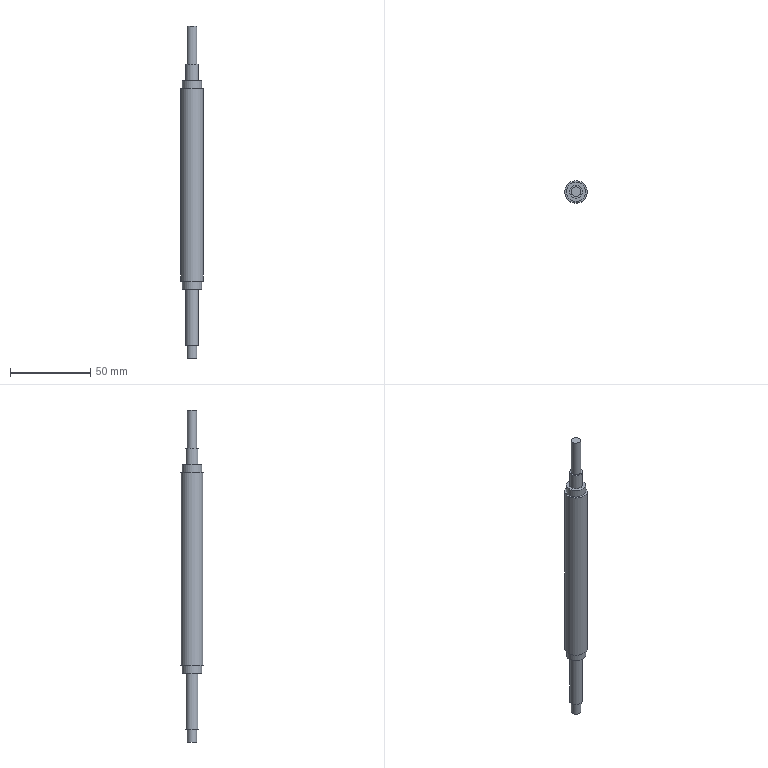Component | NX | Z_AXIS_LEADSCREW | 1 solid | 15 faces | box 14 x 14 x 207 mm | volume 22770 mm3 | plane 8 | cylinder 7 | commonest cylinder face diameters 6 x2 8 x2 12 x2 14 x1
STEP:
#1=CARTESIAN_POINT('',(0.,0.,0.));
#2=DIRECTION('',(0.,0.,1.));
#3=DIRECTION('',(1.,0.,0.));
#4=AXIS2_PLACEMENT_3D('',#1,#2,#3);
#5=CARTESIAN_POINT('',(628.689,-150.302,-1191.));
#6=VERTEX_POINT('',#5);
#7=CARTESIAN_POINT('',(625.689,-150.302,-1191.));
#8=DIRECTION('',(0.,0.,1.));
#9=DIRECTION('',(1.,0.,0.));
#10=AXIS2_PLACEMENT_3D('',#7,#8,#9);
#11=CIRCLE('',#10,3.);
#12=CARTESIAN_POINT('',(625.689,-150.302,-1191.));
#13=DIRECTION('',(0.,0.,1.));
#14=DIRECTION('',(1.,0.,0.));
#15=AXIS2_PLACEMENT_3D('',#12,#13,#14);
#16=PLANE('',#15);
#17=CARTESIAN_POINT('',(0.,0.));
#18=DIRECTION('',(1.,0.));
#19=AXIS2_PLACEMENT_2D('',#17,#18);
#20=CIRCLE('',#19,3.);
#21=(GEOMETRIC_REPRESENTATION_CONTEXT(2)PARAMETRIC_REPRESENTATION_CONTEXT()REPRESENTATION_CONTEXT('',''));
#22=DEFINITIONAL_REPRESENTATION('',(#20),#21);
#23=PCURVE('',#16,#22);
#24=CARTESIAN_POINT('',(625.689,-150.302,-1083.));
#25=DIRECTION('',(0.,0.,1.));
#26=DIRECTION('',(1.,0.,0.));
#27=AXIS2_PLACEMENT_3D('',#24,#25,#26);
#28=CYLINDRICAL_SURFACE('',#27,3.);
#29=CARTESIAN_POINT('',(0.,-108.));
#30=DIRECTION('',(1.,0.));
#31=VECTOR('',#30,1.);
#32=LINE('',#29,#31);
#33=(GEOMETRIC_REPRESENTATION_CONTEXT(2)PARAMETRIC_REPRESENTATION_CONTEXT()REPRESENTATION_CONTEXT('',''));
#34=DEFINITIONAL_REPRESENTATION('',(#32),#33);
#35=PCURVE('',#28,#34);
#36=SURFACE_CURVE('',#11,(#23,#35),.PCURVE_S1.);
#37=EDGE_CURVE('',#6,#6,#36,.T.);
#38=ORIENTED_EDGE('',*,*,#37,.F.);
#39=EDGE_LOOP('',(#38));
#40=FACE_BOUND('',#39,.T.);
#41=ADVANCED_FACE('',(#40),#16,.F.);
#42=CARTESIAN_POINT('',(628.689,-150.302,-984.));
#43=VERTEX_POINT('',#42);
#44=CARTESIAN_POINT('',(625.689,-150.302,-984.));
#45=DIRECTION('',(0.,0.,1.));
#46=DIRECTION('',(1.,0.,0.));
#47=AXIS2_PLACEMENT_3D('',#44,#45,#46);
#48=CIRCLE('',#47,3.);
#49=CARTESIAN_POINT('',(625.689,-150.302,-984.));
#50=DIRECTION('',(0.,0.,1.));
#51=DIRECTION('',(1.,0.,0.));
#52=AXIS2_PLACEMENT_3D('',#49,#50,#51);
#53=PLANE('',#52);
#54=CARTESIAN_POINT('',(0.,0.));
#55=DIRECTION('',(1.,0.));
#56=AXIS2_PLACEMENT_2D('',#54,#55);
#57=CIRCLE('',#56,3.);
#58=(GEOMETRIC_REPRESENTATION_CONTEXT(2)PARAMETRIC_REPRESENTATION_CONTEXT()REPRESENTATION_CONTEXT('',''));
#59=DEFINITIONAL_REPRESENTATION('',(#57),#58);
#60=PCURVE('',#53,#59);
#61=CARTESIAN_POINT('',(625.689,-150.302,-1083.));
#62=DIRECTION('',(0.,0.,1.));
#63=DIRECTION('',(1.,0.,0.));
#64=AXIS2_PLACEMENT_3D('',#61,#62,#63);
#65=CYLINDRICAL_SURFACE('',#64,3.);
#66=CARTESIAN_POINT('',(0.,99.));
#67=DIRECTION('',(1.,0.));
#68=VECTOR('',#67,1.);
#69=LINE('',#66,#68);
#70=(GEOMETRIC_REPRESENTATION_CONTEXT(2)PARAMETRIC_REPRESENTATION_CONTEXT()REPRESENTATION_CONTEXT('',''));
#71=DEFINITIONAL_REPRESENTATION('',(#69),#70);
#72=PCURVE('',#65,#71);
#73=SURFACE_CURVE('',#48,(#60,#72),.PCURVE_S1.);
#74=EDGE_CURVE('',#43,#43,#73,.T.);
#75=ORIENTED_EDGE('',*,*,#74,.T.);
#76=EDGE_LOOP('',(#75));
#77=FACE_BOUND('',#76,.T.);
#78=ADVANCED_FACE('',(#77),#53,.T.);
#79=ORIENTED_EDGE('',*,*,#74,.F.);
#80=CARTESIAN_POINT('',(628.689,-150.302,-1008.));
#81=VERTEX_POINT('',#80);
#82=CARTESIAN_POINT('',(628.689,-150.302,-1008.));
#83=CARTESIAN_POINT('',(628.689,-150.302,-984.));
#84=B_SPLINE_CURVE_WITH_KNOTS('',1,(#82,#83),.UNSPECIFIED.,.F.,.F.,(2,2),(75.,99.),.PIECEWISE_BEZIER_KNOTS.);
#85=CARTESIAN_POINT('',(0.,0.));
#86=DIRECTION('',(0.,1.));
#87=VECTOR('',#86,1.);
#88=LINE('',#85,#87);
#89=(GEOMETRIC_REPRESENTATION_CONTEXT(2)PARAMETRIC_REPRESENTATION_CONTEXT()REPRESENTATION_CONTEXT('',''));
#90=DEFINITIONAL_REPRESENTATION('',(#88),#89);
#91=PCURVE('',#65,#90);
#92=CARTESIAN_POINT('',(6.283,0.));
#93=DIRECTION('',(0.,1.));
#94=VECTOR('',#93,1.);
#95=LINE('',#92,#94);
#96=(GEOMETRIC_REPRESENTATION_CONTEXT(2)PARAMETRIC_REPRESENTATION_CONTEXT()REPRESENTATION_CONTEXT('',''));
#97=DEFINITIONAL_REPRESENTATION('',(#95),#96);
#98=PCURVE('',#65,#97);
#99=SEAM_CURVE('',#84,(#91,#98),.PCURVE_S1.);
#100=EDGE_CURVE('',#81,#43,#99,.T.);
#101=ORIENTED_EDGE('',*,*,#100,.F.);
#102=CARTESIAN_POINT('',(625.689,-150.302,-1008.));
#103=DIRECTION('',(0.,0.,1.));
#104=DIRECTION('',(1.,0.,0.));
#105=AXIS2_PLACEMENT_3D('',#102,#103,#104);
#106=CIRCLE('',#105,3.);
#107=CARTESIAN_POINT('',(0.,75.));
#108=DIRECTION('',(1.,0.));
#109=VECTOR('',#108,1.);
#110=LINE('',#107,#109);
#111=(GEOMETRIC_REPRESENTATION_CONTEXT(2)PARAMETRIC_REPRESENTATION_CONTEXT()REPRESENTATION_CONTEXT('',''));
#112=DEFINITIONAL_REPRESENTATION('',(#110),#111);
#113=PCURVE('',#65,#112);
#114=CARTESIAN_POINT('',(621.689,-150.302,-1008.));
#115=DIRECTION('',(0.,0.,-1.));
#116=DIRECTION('',(-1.,0.,0.));
#117=AXIS2_PLACEMENT_3D('',#114,#115,#116);
#118=PLANE('',#117);
#119=CARTESIAN_POINT('',(-7.,0.));
#120=CARTESIAN_POINT('',(-7.,5.196));
#121=CARTESIAN_POINT('',(-2.5,2.598));
#122=CARTESIAN_POINT('',(2.,0.));
#123=CARTESIAN_POINT('',(-2.5,-2.598));
#124=CARTESIAN_POINT('',(-7.,-5.196));
#125=CARTESIAN_POINT('',(-7.,0.));
#126=(BOUNDED_CURVE()B_SPLINE_CURVE(2,(#119,#120,#121,#122,#123,#124,#125),.UNSPECIFIED.,.T.,.F.)B_SPLINE_CURVE_WITH_KNOTS((1,2,2,2,2,1),(-2.094,0.,2.094,4.189,6.283,8.378),.UNSPECIFIED.)CURVE()GEOMETRIC_REPRESENTATION_ITEM()RATIONAL_B_SPLINE_CURVE((1.,0.5,1.,0.5,1.,0.5,1.))REPRESENTATION_ITEM(''));
#127=(GEOMETRIC_REPRESENTATION_CONTEXT(2)PARAMETRIC_REPRESENTATION_CONTEXT()REPRESENTATION_CONTEXT('',''));
#128=DEFINITIONAL_REPRESENTATION('',(#126),#127);
#129=PCURVE('',#118,#128);
#130=SURFACE_CURVE('',#106,(#113,#129),.PCURVE_S1.);
#131=EDGE_CURVE('',#81,#81,#130,.T.);
#132=ORIENTED_EDGE('',*,*,#131,.T.);
#133=ORIENTED_EDGE('',*,*,#100,.T.);
#134=EDGE_LOOP('',(#79,#101,#132,#133));
#135=FACE_BOUND('',#134,.T.);
#136=ADVANCED_FACE('',(#135),#65,.T.);
#137=ORIENTED_EDGE('',*,*,#131,.F.);
#138=EDGE_LOOP('',(#137));
#139=FACE_BOUND('',#138,.T.);
#140=CARTESIAN_POINT('',(629.689,-150.302,-1008.));
#141=VERTEX_POINT('',#140);
#142=CARTESIAN_POINT('',(625.689,-150.302,-1008.));
#143=DIRECTION('',(0.,0.,1.));
#144=DIRECTION('',(1.,0.,0.));
#145=AXIS2_PLACEMENT_3D('',#142,#143,#144);
#146=CIRCLE('',#145,4.);
#147=CARTESIAN_POINT('',(-8.,0.));
#148=CARTESIAN_POINT('',(-8.,6.928));
#149=CARTESIAN_POINT('',(-2.,3.464));
#150=CARTESIAN_POINT('',(4.,0.));
#151=CARTESIAN_POINT('',(-2.,-3.464));
#152=CARTESIAN_POINT('',(-8.,-6.928));
#153=CARTESIAN_POINT('',(-8.,0.));
#154=(BOUNDED_CURVE()B_SPLINE_CURVE(2,(#147,#148,#149,#150,#151,#152,#153),.UNSPECIFIED.,.T.,.F.)B_SPLINE_CURVE_WITH_KNOTS((1,2,2,2,2,1),(-2.094,0.,2.094,4.189,6.283,8.378),.UNSPECIFIED.)CURVE()GEOMETRIC_REPRESENTATION_ITEM()RATIONAL_B_SPLINE_CURVE((1.,0.5,1.,0.5,1.,0.5,1.))REPRESENTATION_ITEM(''));
#155=(GEOMETRIC_REPRESENTATION_CONTEXT(2)PARAMETRIC_REPRESENTATION_CONTEXT()REPRESENTATION_CONTEXT('',''));
#156=DEFINITIONAL_REPRESENTATION('',(#154),#155);
#157=PCURVE('',#118,#156);
#158=CARTESIAN_POINT('',(625.689,-150.302,-1083.));
#159=DIRECTION('',(0.,0.,1.));
#160=DIRECTION('',(1.,0.,0.));
#161=AXIS2_PLACEMENT_3D('',#158,#159,#160);
#162=CYLINDRICAL_SURFACE('',#161,4.);
#163=CARTESIAN_POINT('',(0.,75.));
#164=DIRECTION('',(1.,0.));
#165=VECTOR('',#164,1.);
#166=LINE('',#163,#165);
#167=(GEOMETRIC_REPRESENTATION_CONTEXT(2)PARAMETRIC_REPRESENTATION_CONTEXT()REPRESENTATION_CONTEXT('',''));
#168=DEFINITIONAL_REPRESENTATION('',(#166),#167);
#169=PCURVE('',#162,#168);
#170=SURFACE_CURVE('',#146,(#157,#169),.PCURVE_S1.);
#171=EDGE_CURVE('',#141,#141,#170,.T.);
#172=ORIENTED_EDGE('',*,*,#171,.T.);
#173=EDGE_LOOP('',(#172));
#174=FACE_BOUND('',#173,.T.);
#175=ADVANCED_FACE('',(#139,#174),#118,.F.);
#176=ORIENTED_EDGE('',*,*,#171,.F.);
#177=CARTESIAN_POINT('',(629.689,-150.302,-1018.));
#178=VERTEX_POINT('',#177);
#179=CARTESIAN_POINT('',(629.689,-150.302,-1018.));
#180=CARTESIAN_POINT('',(629.689,-150.302,-1008.));
#181=B_SPLINE_CURVE_WITH_KNOTS('',1,(#179,#180),.UNSPECIFIED.,.F.,.F.,(2,2),(65.,75.),.PIECEWISE_BEZIER_KNOTS.);
#182=CARTESIAN_POINT('',(0.,0.));
#183=DIRECTION('',(0.,1.));
#184=VECTOR('',#183,1.);
#185=LINE('',#182,#184);
#186=(GEOMETRIC_REPRESENTATION_CONTEXT(2)PARAMETRIC_REPRESENTATION_CONTEXT()REPRESENTATION_CONTEXT('',''));
#187=DEFINITIONAL_REPRESENTATION('',(#185),#186);
#188=PCURVE('',#162,#187);
#189=CARTESIAN_POINT('',(6.283,0.));
#190=DIRECTION('',(0.,1.));
#191=VECTOR('',#190,1.);
#192=LINE('',#189,#191);
#193=(GEOMETRIC_REPRESENTATION_CONTEXT(2)PARAMETRIC_REPRESENTATION_CONTEXT()REPRESENTATION_CONTEXT('',''));
#194=DEFINITIONAL_REPRESENTATION('',(#192),#193);
#195=PCURVE('',#162,#194);
#196=SEAM_CURVE('',#181,(#188,#195),.PCURVE_S1.);
#197=EDGE_CURVE('',#178,#141,#196,.T.);
#198=ORIENTED_EDGE('',*,*,#197,.F.);
#199=CARTESIAN_POINT('',(625.689,-150.302,-1018.));
#200=DIRECTION('',(0.,0.,1.));
#201=DIRECTION('',(1.,0.,0.));
#202=AXIS2_PLACEMENT_3D('',#199,#200,#201);
#203=CIRCLE('',#202,4.);
#204=CARTESIAN_POINT('',(0.,65.));
#205=DIRECTION('',(1.,0.));
#206=VECTOR('',#205,1.);
#207=LINE('',#204,#206);
#208=(GEOMETRIC_REPRESENTATION_CONTEXT(2)PARAMETRIC_REPRESENTATION_CONTEXT()REPRESENTATION_CONTEXT('',''));
#209=DEFINITIONAL_REPRESENTATION('',(#207),#208);
#210=PCURVE('',#162,#209);
#211=CARTESIAN_POINT('',(619.689,-150.302,-1018.));
#212=DIRECTION('',(0.,0.,-1.));
#213=DIRECTION('',(-1.,0.,0.));
#214=AXIS2_PLACEMENT_3D('',#211,#212,#213);
#215=PLANE('',#214);
#216=CARTESIAN_POINT('',(-10.,0.));
#217=CARTESIAN_POINT('',(-10.,6.928));
#218=CARTESIAN_POINT('',(-4.,3.464));
#219=CARTESIAN_POINT('',(2.,0.));
#220=CARTESIAN_POINT('',(-4.,-3.464));
#221=CARTESIAN_POINT('',(-10.,-6.928));
#222=CARTESIAN_POINT('',(-10.,0.));
#223=(BOUNDED_CURVE()B_SPLINE_CURVE(2,(#216,#217,#218,#219,#220,#221,#222),.UNSPECIFIED.,.T.,.F.)B_SPLINE_CURVE_WITH_KNOTS((1,2,2,2,2,1),(-2.094,0.,2.094,4.189,6.283,8.378),.UNSPECIFIED.)CURVE()GEOMETRIC_REPRESENTATION_ITEM()RATIONAL_B_SPLINE_CURVE((1.,0.5,1.,0.5,1.,0.5,1.))REPRESENTATION_ITEM(''));
#224=(GEOMETRIC_REPRESENTATION_CONTEXT(2)PARAMETRIC_REPRESENTATION_CONTEXT()REPRESENTATION_CONTEXT('',''));
#225=DEFINITIONAL_REPRESENTATION('',(#223),#224);
#226=PCURVE('',#215,#225);
#227=SURFACE_CURVE('',#203,(#210,#226),.PCURVE_S1.);
#228=EDGE_CURVE('',#178,#178,#227,.T.);
#229=ORIENTED_EDGE('',*,*,#228,.T.);
#230=ORIENTED_EDGE('',*,*,#197,.T.);
#231=EDGE_LOOP('',(#176,#198,#229,#230));
#232=FACE_BOUND('',#231,.T.);
#233=ADVANCED_FACE('',(#232),#162,.T.);
#234=ORIENTED_EDGE('',*,*,#228,.F.);
#235=EDGE_LOOP('',(#234));
#236=FACE_BOUND('',#235,.T.);
#237=CARTESIAN_POINT('',(631.689,-150.302,-1018.));
#238=VERTEX_POINT('',#237);
#239=CARTESIAN_POINT('',(625.689,-150.302,-1018.));
#240=DIRECTION('',(0.,0.,1.));
#241=DIRECTION('',(1.,0.,0.));
#242=AXIS2_PLACEMENT_3D('',#239,#240,#241);
#243=CIRCLE('',#242,6.);
#244=CARTESIAN_POINT('',(-12.,0.));
#245=CARTESIAN_POINT('',(-12.,10.392));
#246=CARTESIAN_POINT('',(-3.,5.196));
#247=CARTESIAN_POINT('',(6.,0.));
#248=CARTESIAN_POINT('',(-3.,-5.196));
#249=CARTESIAN_POINT('',(-12.,-10.392));
#250=CARTESIAN_POINT('',(-12.,0.));
#251=(BOUNDED_CURVE()B_SPLINE_CURVE(2,(#244,#245,#246,#247,#248,#249,#250),.UNSPECIFIED.,.T.,.F.)B_SPLINE_CURVE_WITH_KNOTS((1,2,2,2,2,1),(-2.094,0.,2.094,4.189,6.283,8.378),.UNSPECIFIED.)CURVE()GEOMETRIC_REPRESENTATION_ITEM()RATIONAL_B_SPLINE_CURVE((1.,0.5,1.,0.5,1.,0.5,1.))REPRESENTATION_ITEM(''));
#252=(GEOMETRIC_REPRESENTATION_CONTEXT(2)PARAMETRIC_REPRESENTATION_CONTEXT()REPRESENTATION_CONTEXT('',''));
#253=DEFINITIONAL_REPRESENTATION('',(#251),#252);
#254=PCURVE('',#215,#253);
#255=CARTESIAN_POINT('',(625.689,-150.302,-1083.));
#256=DIRECTION('',(0.,0.,1.));
#257=DIRECTION('',(1.,0.,0.));
#258=AXIS2_PLACEMENT_3D('',#255,#256,#257);
#259=CYLINDRICAL_SURFACE('',#258,6.);
#260=CARTESIAN_POINT('',(0.,65.));
#261=DIRECTION('',(1.,0.));
#262=VECTOR('',#261,1.);
#263=LINE('',#260,#262);
#264=(GEOMETRIC_REPRESENTATION_CONTEXT(2)PARAMETRIC_REPRESENTATION_CONTEXT()REPRESENTATION_CONTEXT('',''));
#265=DEFINITIONAL_REPRESENTATION('',(#263),#264);
#266=PCURVE('',#259,#265);
#267=SURFACE_CURVE('',#243,(#254,#266),.PCURVE_S1.);
#268=EDGE_CURVE('',#238,#238,#267,.T.);
#269=ORIENTED_EDGE('',*,*,#268,.T.);
#270=EDGE_LOOP('',(#269));
#271=FACE_BOUND('',#270,.T.);
#272=ADVANCED_FACE('',(#236,#271),#215,.F.);
#273=ORIENTED_EDGE('',*,*,#268,.F.);
#274=CARTESIAN_POINT('',(631.689,-150.302,-1023.));
#275=VERTEX_POINT('',#274);
#276=CARTESIAN_POINT('',(631.689,-150.302,-1023.));
#277=CARTESIAN_POINT('',(631.689,-150.302,-1018.));
#278=B_SPLINE_CURVE_WITH_KNOTS('',1,(#276,#277),.UNSPECIFIED.,.F.,.F.,(2,2),(60.,65.),.PIECEWISE_BEZIER_KNOTS.);
#279=CARTESIAN_POINT('',(0.,0.));
#280=DIRECTION('',(0.,1.));
#281=VECTOR('',#280,1.);
#282=LINE('',#279,#281);
#283=(GEOMETRIC_REPRESENTATION_CONTEXT(2)PARAMETRIC_REPRESENTATION_CONTEXT()REPRESENTATION_CONTEXT('',''));
#284=DEFINITIONAL_REPRESENTATION('',(#282),#283);
#285=PCURVE('',#259,#284);
#286=CARTESIAN_POINT('',(6.283,0.));
#287=DIRECTION('',(0.,1.));
#288=VECTOR('',#287,1.);
#289=LINE('',#286,#288);
#290=(GEOMETRIC_REPRESENTATION_CONTEXT(2)PARAMETRIC_REPRESENTATION_CONTEXT()REPRESENTATION_CONTEXT('',''));
#291=DEFINITIONAL_REPRESENTATION('',(#289),#290);
#292=PCURVE('',#259,#291);
#293=SEAM_CURVE('',#278,(#285,#292),.PCURVE_S1.);
#294=EDGE_CURVE('',#275,#238,#293,.T.);
#295=ORIENTED_EDGE('',*,*,#294,.F.);
#296=CARTESIAN_POINT('',(625.689,-150.302,-1023.));
#297=DIRECTION('',(0.,0.,1.));
#298=DIRECTION('',(1.,0.,0.));
#299=AXIS2_PLACEMENT_3D('',#296,#297,#298);
#300=CIRCLE('',#299,6.);
#301=CARTESIAN_POINT('',(0.,60.));
#302=DIRECTION('',(1.,0.));
#303=VECTOR('',#302,1.);
#304=LINE('',#301,#303);
#305=(GEOMETRIC_REPRESENTATION_CONTEXT(2)PARAMETRIC_REPRESENTATION_CONTEXT()REPRESENTATION_CONTEXT('',''));
#306=DEFINITIONAL_REPRESENTATION('',(#304),#305);
#307=PCURVE('',#259,#306);
#308=CARTESIAN_POINT('',(618.689,-150.302,-1023.));
#309=DIRECTION('',(0.,0.,-1.));
#310=DIRECTION('',(-1.,0.,0.));
#311=AXIS2_PLACEMENT_3D('',#308,#309,#310);
#312=PLANE('',#311);
#313=CARTESIAN_POINT('',(-13.,0.));
#314=CARTESIAN_POINT('',(-13.,10.392));
#315=CARTESIAN_POINT('',(-4.,5.196));
#316=CARTESIAN_POINT('',(5.,0.));
#317=CARTESIAN_POINT('',(-4.,-5.196));
#318=CARTESIAN_POINT('',(-13.,-10.392));
#319=CARTESIAN_POINT('',(-13.,0.));
#320=(BOUNDED_CURVE()B_SPLINE_CURVE(2,(#313,#314,#315,#316,#317,#318,#319),.UNSPECIFIED.,.T.,.F.)B_SPLINE_CURVE_WITH_KNOTS((1,2,2,2,2,1),(-2.094,0.,2.094,4.189,6.283,8.378),.UNSPECIFIED.)CURVE()GEOMETRIC_REPRESENTATION_ITEM()RATIONAL_B_SPLINE_CURVE((1.,0.5,1.,0.5,1.,0.5,1.))REPRESENTATION_ITEM(''));
#321=(GEOMETRIC_REPRESENTATION_CONTEXT(2)PARAMETRIC_REPRESENTATION_CONTEXT()REPRESENTATION_CONTEXT('',''));
#322=DEFINITIONAL_REPRESENTATION('',(#320),#321);
#323=PCURVE('',#312,#322);
#324=SURFACE_CURVE('',#300,(#307,#323),.PCURVE_S1.);
#325=EDGE_CURVE('',#275,#275,#324,.T.);
#326=ORIENTED_EDGE('',*,*,#325,.T.);
#327=ORIENTED_EDGE('',*,*,#294,.T.);
#328=EDGE_LOOP('',(#273,#295,#326,#327));
#329=FACE_BOUND('',#328,.T.);
#330=ADVANCED_FACE('',(#329),#259,.T.);
#331=ORIENTED_EDGE('',*,*,#325,.F.);
#332=EDGE_LOOP('',(#331));
#333=FACE_BOUND('',#332,.T.);
#334=CARTESIAN_POINT('',(632.689,-150.302,-1023.));
#335=VERTEX_POINT('',#334);
#336=CARTESIAN_POINT('',(625.689,-150.302,-1023.));
#337=DIRECTION('',(0.,0.,1.));
#338=DIRECTION('',(1.,0.,0.));
#339=AXIS2_PLACEMENT_3D('',#336,#337,#338);
#340=CIRCLE('',#339,7.);
#341=CARTESIAN_POINT('',(-14.,0.));
#342=CARTESIAN_POINT('',(-14.,12.124));
#343=CARTESIAN_POINT('',(-3.5,6.062));
#344=CARTESIAN_POINT('',(7.,0.));
#345=CARTESIAN_POINT('',(-3.5,-6.062));
#346=CARTESIAN_POINT('',(-14.,-12.124));
#347=CARTESIAN_POINT('',(-14.,0.));
#348=(BOUNDED_CURVE()B_SPLINE_CURVE(2,(#341,#342,#343,#344,#345,#346,#347),.UNSPECIFIED.,.T.,.F.)B_SPLINE_CURVE_WITH_KNOTS((1,2,2,2,2,1),(-2.094,0.,2.094,4.189,6.283,8.378),.UNSPECIFIED.)CURVE()GEOMETRIC_REPRESENTATION_ITEM()RATIONAL_B_SPLINE_CURVE((1.,0.5,1.,0.5,1.,0.5,1.))REPRESENTATION_ITEM(''));
#349=(GEOMETRIC_REPRESENTATION_CONTEXT(2)PARAMETRIC_REPRESENTATION_CONTEXT()REPRESENTATION_CONTEXT('',''));
#350=DEFINITIONAL_REPRESENTATION('',(#348),#349);
#351=PCURVE('',#312,#350);
#352=CARTESIAN_POINT('',(625.689,-150.302,-1083.));
#353=DIRECTION('',(0.,0.,1.));
#354=DIRECTION('',(1.,0.,0.));
#355=AXIS2_PLACEMENT_3D('',#352,#353,#354);
#356=CYLINDRICAL_SURFACE('',#355,7.);
#357=CARTESIAN_POINT('',(0.,60.));
#358=DIRECTION('',(1.,0.));
#359=VECTOR('',#358,1.);
#360=LINE('',#357,#359);
#361=(GEOMETRIC_REPRESENTATION_CONTEXT(2)PARAMETRIC_REPRESENTATION_CONTEXT()REPRESENTATION_CONTEXT('',''));
#362=DEFINITIONAL_REPRESENTATION('',(#360),#361);
#363=PCURVE('',#356,#362);
#364=SURFACE_CURVE('',#340,(#351,#363),.PCURVE_S1.);
#365=EDGE_CURVE('',#335,#335,#364,.T.);
#366=ORIENTED_EDGE('',*,*,#365,.T.);
#367=EDGE_LOOP('',(#366));
#368=FACE_BOUND('',#367,.T.);
#369=ADVANCED_FACE('',(#333,#368),#312,.F.);
#370=ORIENTED_EDGE('',*,*,#365,.F.);
#371=CARTESIAN_POINT('',(632.689,-150.302,-1143.));
#372=VERTEX_POINT('',#371);
#373=CARTESIAN_POINT('',(632.689,-150.302,-1143.));
#374=CARTESIAN_POINT('',(632.689,-150.302,-1023.));
#375=B_SPLINE_CURVE_WITH_KNOTS('',1,(#373,#374),.UNSPECIFIED.,.F.,.F.,(2,2),(-60.,60.),.PIECEWISE_BEZIER_KNOTS.);
#376=CARTESIAN_POINT('',(0.,0.));
#377=DIRECTION('',(0.,1.));
#378=VECTOR('',#377,1.);
#379=LINE('',#376,#378);
#380=(GEOMETRIC_REPRESENTATION_CONTEXT(2)PARAMETRIC_REPRESENTATION_CONTEXT()REPRESENTATION_CONTEXT('',''));
#381=DEFINITIONAL_REPRESENTATION('',(#379),#380);
#382=PCURVE('',#356,#381);
#383=CARTESIAN_POINT('',(6.283,0.));
#384=DIRECTION('',(0.,1.));
#385=VECTOR('',#384,1.);
#386=LINE('',#383,#385);
#387=(GEOMETRIC_REPRESENTATION_CONTEXT(2)PARAMETRIC_REPRESENTATION_CONTEXT()REPRESENTATION_CONTEXT('',''));
#388=DEFINITIONAL_REPRESENTATION('',(#386),#387);
#389=PCURVE('',#356,#388);
#390=SEAM_CURVE('',#375,(#382,#389),.PCURVE_S1.);
#391=EDGE_CURVE('',#372,#335,#390,.T.);
#392=ORIENTED_EDGE('',*,*,#391,.F.);
#393=CARTESIAN_POINT('',(625.689,-150.302,-1143.));
#394=DIRECTION('',(0.,0.,1.));
#395=DIRECTION('',(1.,0.,0.));
#396=AXIS2_PLACEMENT_3D('',#393,#394,#395);
#397=CIRCLE('',#396,7.);
#398=CARTESIAN_POINT('',(0.,-60.));
#399=DIRECTION('',(1.,0.));
#400=VECTOR('',#399,1.);
#401=LINE('',#398,#400);
#402=(GEOMETRIC_REPRESENTATION_CONTEXT(2)PARAMETRIC_REPRESENTATION_CONTEXT()REPRESENTATION_CONTEXT('',''));
#403=DEFINITIONAL_REPRESENTATION('',(#401),#402);
#404=PCURVE('',#356,#403);
#405=CARTESIAN_POINT('',(619.689,-150.302,-1143.));
#406=DIRECTION('',(0.,0.,1.));
#407=DIRECTION('',(1.,0.,0.));
#408=AXIS2_PLACEMENT_3D('',#405,#406,#407);
#409=PLANE('',#408);
#410=CARTESIAN_POINT('',(6.,0.));
#411=DIRECTION('',(1.,0.));
#412=AXIS2_PLACEMENT_2D('',#410,#411);
#413=CIRCLE('',#412,7.);
#414=(GEOMETRIC_REPRESENTATION_CONTEXT(2)PARAMETRIC_REPRESENTATION_CONTEXT()REPRESENTATION_CONTEXT('',''));
#415=DEFINITIONAL_REPRESENTATION('',(#413),#414);
#416=PCURVE('',#409,#415);
#417=SURFACE_CURVE('',#397,(#404,#416),.PCURVE_S1.);
#418=EDGE_CURVE('',#372,#372,#417,.T.);
#419=ORIENTED_EDGE('',*,*,#418,.T.);
#420=ORIENTED_EDGE('',*,*,#391,.T.);
#421=EDGE_LOOP('',(#370,#392,#419,#420));
#422=FACE_BOUND('',#421,.T.);
#423=ADVANCED_FACE('',(#422),#356,.T.);
#424=ORIENTED_EDGE('',*,*,#418,.F.);
#425=EDGE_LOOP('',(#424));
#426=FACE_BOUND('',#425,.T.);
#427=CARTESIAN_POINT('',(631.689,-150.302,-1143.));
#428=VERTEX_POINT('',#427);
#429=CARTESIAN_POINT('',(625.689,-150.302,-1143.));
#430=DIRECTION('',(0.,0.,1.));
#431=DIRECTION('',(1.,0.,0.));
#432=AXIS2_PLACEMENT_3D('',#429,#430,#431);
#433=CIRCLE('',#432,6.);
#434=CARTESIAN_POINT('',(6.,0.));
#435=DIRECTION('',(1.,0.));
#436=AXIS2_PLACEMENT_2D('',#434,#435);
#437=CIRCLE('',#436,6.);
#438=(GEOMETRIC_REPRESENTATION_CONTEXT(2)PARAMETRIC_REPRESENTATION_CONTEXT()REPRESENTATION_CONTEXT('',''));
#439=DEFINITIONAL_REPRESENTATION('',(#437),#438);
#440=PCURVE('',#409,#439);
#441=CARTESIAN_POINT('',(625.689,-150.302,-1083.));
#442=DIRECTION('',(0.,0.,1.));
#443=DIRECTION('',(1.,0.,0.));
#444=AXIS2_PLACEMENT_3D('',#441,#442,#443);
#445=CYLINDRICAL_SURFACE('',#444,6.);
#446=CARTESIAN_POINT('',(0.,-60.));
#447=DIRECTION('',(1.,0.));
#448=VECTOR('',#447,1.);
#449=LINE('',#446,#448);
#450=(GEOMETRIC_REPRESENTATION_CONTEXT(2)PARAMETRIC_REPRESENTATION_CONTEXT()REPRESENTATION_CONTEXT('',''));
#451=DEFINITIONAL_REPRESENTATION('',(#449),#450);
#452=PCURVE('',#445,#451);
#453=SURFACE_CURVE('',#433,(#440,#452),.PCURVE_S1.);
#454=EDGE_CURVE('',#428,#428,#453,.T.);
#455=ORIENTED_EDGE('',*,*,#454,.T.);
#456=EDGE_LOOP('',(#455));
#457=FACE_BOUND('',#456,.T.);
#458=ADVANCED_FACE('',(#426,#457),#409,.F.);
#459=ORIENTED_EDGE('',*,*,#454,.F.);
#460=CARTESIAN_POINT('',(631.689,-150.302,-1148.));
#461=VERTEX_POINT('',#460);
#462=CARTESIAN_POINT('',(631.689,-150.302,-1148.));
#463=CARTESIAN_POINT('',(631.689,-150.302,-1143.));
#464=B_SPLINE_CURVE_WITH_KNOTS('',1,(#462,#463),.UNSPECIFIED.,.F.,.F.,(2,2),(-65.,-60.),.PIECEWISE_BEZIER_KNOTS.);
#465=CARTESIAN_POINT('',(0.,0.));
#466=DIRECTION('',(0.,1.));
#467=VECTOR('',#466,1.);
#468=LINE('',#465,#467);
#469=(GEOMETRIC_REPRESENTATION_CONTEXT(2)PARAMETRIC_REPRESENTATION_CONTEXT()REPRESENTATION_CONTEXT('',''));
#470=DEFINITIONAL_REPRESENTATION('',(#468),#469);
#471=PCURVE('',#445,#470);
#472=CARTESIAN_POINT('',(6.283,0.));
#473=DIRECTION('',(0.,1.));
#474=VECTOR('',#473,1.);
#475=LINE('',#472,#474);
#476=(GEOMETRIC_REPRESENTATION_CONTEXT(2)PARAMETRIC_REPRESENTATION_CONTEXT()REPRESENTATION_CONTEXT('',''));
#477=DEFINITIONAL_REPRESENTATION('',(#475),#476);
#478=PCURVE('',#445,#477);
#479=SEAM_CURVE('',#464,(#471,#478),.PCURVE_S1.);
#480=EDGE_CURVE('',#461,#428,#479,.T.);
#481=ORIENTED_EDGE('',*,*,#480,.F.);
#482=CARTESIAN_POINT('',(625.689,-150.302,-1148.));
#483=DIRECTION('',(0.,0.,1.));
#484=DIRECTION('',(1.,0.,0.));
#485=AXIS2_PLACEMENT_3D('',#482,#483,#484);
#486=CIRCLE('',#485,6.);
#487=CARTESIAN_POINT('',(0.,-65.));
#488=DIRECTION('',(1.,0.));
#489=VECTOR('',#488,1.);
#490=LINE('',#487,#489);
#491=(GEOMETRIC_REPRESENTATION_CONTEXT(2)PARAMETRIC_REPRESENTATION_CONTEXT()REPRESENTATION_CONTEXT('',''));
#492=DEFINITIONAL_REPRESENTATION('',(#490),#491);
#493=PCURVE('',#445,#492);
#494=CARTESIAN_POINT('',(621.689,-150.302,-1148.));
#495=DIRECTION('',(0.,0.,1.));
#496=DIRECTION('',(1.,0.,0.));
#497=AXIS2_PLACEMENT_3D('',#494,#495,#496);
#498=PLANE('',#497);
#499=CARTESIAN_POINT('',(4.,0.));
#500=DIRECTION('',(1.,0.));
#501=AXIS2_PLACEMENT_2D('',#499,#500);
#502=CIRCLE('',#501,6.);
#503=(GEOMETRIC_REPRESENTATION_CONTEXT(2)PARAMETRIC_REPRESENTATION_CONTEXT()REPRESENTATION_CONTEXT('',''));
#504=DEFINITIONAL_REPRESENTATION('',(#502),#503);
#505=PCURVE('',#498,#504);
#506=SURFACE_CURVE('',#486,(#493,#505),.PCURVE_S1.);
#507=EDGE_CURVE('',#461,#461,#506,.T.);
#508=ORIENTED_EDGE('',*,*,#507,.T.);
#509=ORIENTED_EDGE('',*,*,#480,.T.);
#510=EDGE_LOOP('',(#459,#481,#508,#509));
#511=FACE_BOUND('',#510,.T.);
#512=ADVANCED_FACE('',(#511),#445,.T.);
#513=ORIENTED_EDGE('',*,*,#507,.F.);
#514=EDGE_LOOP('',(#513));
#515=FACE_BOUND('',#514,.T.);
#516=CARTESIAN_POINT('',(629.689,-150.302,-1148.));
#517=VERTEX_POINT('',#516);
#518=CARTESIAN_POINT('',(625.689,-150.302,-1148.));
#519=DIRECTION('',(0.,0.,1.));
#520=DIRECTION('',(1.,0.,0.));
#521=AXIS2_PLACEMENT_3D('',#518,#519,#520);
#522=CIRCLE('',#521,4.);
#523=CARTESIAN_POINT('',(4.,0.));
#524=DIRECTION('',(1.,0.));
#525=AXIS2_PLACEMENT_2D('',#523,#524);
#526=CIRCLE('',#525,4.);
#527=(GEOMETRIC_REPRESENTATION_CONTEXT(2)PARAMETRIC_REPRESENTATION_CONTEXT()REPRESENTATION_CONTEXT('',''));
#528=DEFINITIONAL_REPRESENTATION('',(#526),#527);
#529=PCURVE('',#498,#528);
#530=CARTESIAN_POINT('',(625.689,-150.302,-1083.));
#531=DIRECTION('',(0.,0.,1.));
#532=DIRECTION('',(1.,0.,0.));
#533=AXIS2_PLACEMENT_3D('',#530,#531,#532);
#534=CYLINDRICAL_SURFACE('',#533,4.);
#535=CARTESIAN_POINT('',(0.,-65.));
#536=DIRECTION('',(1.,0.));
#537=VECTOR('',#536,1.);
#538=LINE('',#535,#537);
#539=(GEOMETRIC_REPRESENTATION_CONTEXT(2)PARAMETRIC_REPRESENTATION_CONTEXT()REPRESENTATION_CONTEXT('',''));
#540=DEFINITIONAL_REPRESENTATION('',(#538),#539);
#541=PCURVE('',#534,#540);
#542=SURFACE_CURVE('',#522,(#529,#541),.PCURVE_S1.);
#543=EDGE_CURVE('',#517,#517,#542,.T.);
#544=ORIENTED_EDGE('',*,*,#543,.T.);
#545=EDGE_LOOP('',(#544));
#546=FACE_BOUND('',#545,.T.);
#547=ADVANCED_FACE('',(#515,#546),#498,.F.);
#548=ORIENTED_EDGE('',*,*,#543,.F.);
#549=CARTESIAN_POINT('',(629.689,-150.302,-1183.));
#550=VERTEX_POINT('',#549);
#551=CARTESIAN_POINT('',(629.689,-150.302,-1183.));
#552=CARTESIAN_POINT('',(629.689,-150.302,-1148.));
#553=B_SPLINE_CURVE_WITH_KNOTS('',1,(#551,#552),.UNSPECIFIED.,.F.,.F.,(2,2),(-100.,-65.),.PIECEWISE_BEZIER_KNOTS.);
#554=CARTESIAN_POINT('',(0.,0.));
#555=DIRECTION('',(0.,1.));
#556=VECTOR('',#555,1.);
#557=LINE('',#554,#556);
#558=(GEOMETRIC_REPRESENTATION_CONTEXT(2)PARAMETRIC_REPRESENTATION_CONTEXT()REPRESENTATION_CONTEXT('',''));
#559=DEFINITIONAL_REPRESENTATION('',(#557),#558);
#560=PCURVE('',#534,#559);
#561=CARTESIAN_POINT('',(6.283,0.));
#562=DIRECTION('',(0.,1.));
#563=VECTOR('',#562,1.);
#564=LINE('',#561,#563);
#565=(GEOMETRIC_REPRESENTATION_CONTEXT(2)PARAMETRIC_REPRESENTATION_CONTEXT()REPRESENTATION_CONTEXT('',''));
#566=DEFINITIONAL_REPRESENTATION('',(#564),#565);
#567=PCURVE('',#534,#566);
#568=SEAM_CURVE('',#553,(#560,#567),.PCURVE_S1.);
#569=EDGE_CURVE('',#550,#517,#568,.T.);
#570=ORIENTED_EDGE('',*,*,#569,.F.);
#571=CARTESIAN_POINT('',(625.689,-150.302,-1183.));
#572=DIRECTION('',(0.,0.,1.));
#573=DIRECTION('',(1.,0.,0.));
#574=AXIS2_PLACEMENT_3D('',#571,#572,#573);
#575=CIRCLE('',#574,4.);
#576=CARTESIAN_POINT('',(0.,-100.));
#577=DIRECTION('',(1.,0.));
#578=VECTOR('',#577,1.);
#579=LINE('',#576,#578);
#580=(GEOMETRIC_REPRESENTATION_CONTEXT(2)PARAMETRIC_REPRESENTATION_CONTEXT()REPRESENTATION_CONTEXT('',''));
#581=DEFINITIONAL_REPRESENTATION('',(#579),#580);
#582=PCURVE('',#534,#581);
#583=CARTESIAN_POINT('',(622.689,-150.302,-1183.));
#584=DIRECTION('',(0.,0.,1.));
#585=DIRECTION('',(1.,0.,0.));
#586=AXIS2_PLACEMENT_3D('',#583,#584,#585);
#587=PLANE('',#586);
#588=CARTESIAN_POINT('',(3.,0.));
#589=DIRECTION('',(1.,0.));
#590=AXIS2_PLACEMENT_2D('',#588,#589);
#591=CIRCLE('',#590,4.);
#592=(GEOMETRIC_REPRESENTATION_CONTEXT(2)PARAMETRIC_REPRESENTATION_CONTEXT()REPRESENTATION_CONTEXT('',''));
#593=DEFINITIONAL_REPRESENTATION('',(#591),#592);
#594=PCURVE('',#587,#593);
#595=SURFACE_CURVE('',#575,(#582,#594),.PCURVE_S1.);
#596=EDGE_CURVE('',#550,#550,#595,.T.);
#597=ORIENTED_EDGE('',*,*,#596,.T.);
#598=ORIENTED_EDGE('',*,*,#569,.T.);
#599=EDGE_LOOP('',(#548,#570,#597,#598));
#600=FACE_BOUND('',#599,.T.);
#601=ADVANCED_FACE('',(#600),#534,.T.);
#602=ORIENTED_EDGE('',*,*,#596,.F.);
#603=EDGE_LOOP('',(#602));
#604=FACE_BOUND('',#603,.T.);
#605=CARTESIAN_POINT('',(628.689,-150.302,-1183.));
#606=VERTEX_POINT('',#605);
#607=CARTESIAN_POINT('',(625.689,-150.302,-1183.));
#608=DIRECTION('',(0.,0.,1.));
#609=DIRECTION('',(1.,0.,0.));
#610=AXIS2_PLACEMENT_3D('',#607,#608,#609);
#611=CIRCLE('',#610,3.);
#612=CARTESIAN_POINT('',(3.,0.));
#613=DIRECTION('',(1.,0.));
#614=AXIS2_PLACEMENT_2D('',#612,#613);
#615=CIRCLE('',#614,3.);
#616=(GEOMETRIC_REPRESENTATION_CONTEXT(2)PARAMETRIC_REPRESENTATION_CONTEXT()REPRESENTATION_CONTEXT('',''));
#617=DEFINITIONAL_REPRESENTATION('',(#615),#616);
#618=PCURVE('',#587,#617);
#619=CARTESIAN_POINT('',(0.,-100.));
#620=DIRECTION('',(1.,0.));
#621=VECTOR('',#620,1.);
#622=LINE('',#619,#621);
#623=(GEOMETRIC_REPRESENTATION_CONTEXT(2)PARAMETRIC_REPRESENTATION_CONTEXT()REPRESENTATION_CONTEXT('',''));
#624=DEFINITIONAL_REPRESENTATION('',(#622),#623);
#625=PCURVE('',#28,#624);
#626=SURFACE_CURVE('',#611,(#618,#625),.PCURVE_S1.);
#627=EDGE_CURVE('',#606,#606,#626,.T.);
#628=ORIENTED_EDGE('',*,*,#627,.T.);
#629=EDGE_LOOP('',(#628));
#630=FACE_BOUND('',#629,.T.);
#631=ADVANCED_FACE('',(#604,#630),#587,.F.);
#632=ORIENTED_EDGE('',*,*,#627,.F.);
#633=CARTESIAN_POINT('',(628.689,-150.302,-1191.));
#634=CARTESIAN_POINT('',(628.689,-150.302,-1183.));
#635=B_SPLINE_CURVE_WITH_KNOTS('',1,(#633,#634),.UNSPECIFIED.,.F.,.F.,(2,2),(-108.,-100.),.PIECEWISE_BEZIER_KNOTS.);
#636=CARTESIAN_POINT('',(0.,0.));
#637=DIRECTION('',(0.,1.));
#638=VECTOR('',#637,1.);
#639=LINE('',#636,#638);
#640=(GEOMETRIC_REPRESENTATION_CONTEXT(2)PARAMETRIC_REPRESENTATION_CONTEXT()REPRESENTATION_CONTEXT('',''));
#641=DEFINITIONAL_REPRESENTATION('',(#639),#640);
#642=PCURVE('',#28,#641);
#643=CARTESIAN_POINT('',(6.283,0.));
#644=DIRECTION('',(0.,1.));
#645=VECTOR('',#644,1.);
#646=LINE('',#643,#645);
#647=(GEOMETRIC_REPRESENTATION_CONTEXT(2)PARAMETRIC_REPRESENTATION_CONTEXT()REPRESENTATION_CONTEXT('',''));
#648=DEFINITIONAL_REPRESENTATION('',(#646),#647);
#649=PCURVE('',#28,#648);
#650=SEAM_CURVE('',#635,(#642,#649),.PCURVE_S1.);
#651=EDGE_CURVE('',#6,#606,#650,.T.);
#652=ORIENTED_EDGE('',*,*,#651,.F.);
#653=ORIENTED_EDGE('',*,*,#37,.T.);
#654=ORIENTED_EDGE('',*,*,#651,.T.);
#655=EDGE_LOOP('',(#632,#652,#653,#654));
#656=FACE_BOUND('',#655,.T.);
#657=ADVANCED_FACE('',(#656),#28,.T.);
#658=CLOSED_SHELL('',(#41,#78,#136,#175,#233,#272,#330,#369,#423,#458,#512,#547,#601,#631,#657));
#659=MANIFOLD_SOLID_BREP('',#658);
#660=(LENGTH_UNIT()NAMED_UNIT(*)SI_UNIT(.MILLI.,.METRE.));
#661=UNCERTAINTY_MEASURE_WITH_UNIT(LENGTH_MEASURE(0.00001),#660,'','');
#662=(NAMED_UNIT(*)PLANE_ANGLE_UNIT()SI_UNIT($,.RADIAN.));
#663=(NAMED_UNIT(*)SI_UNIT($,.STERADIAN.)SOLID_ANGLE_UNIT());
#664=(GEOMETRIC_REPRESENTATION_CONTEXT(3)GLOBAL_UNCERTAINTY_ASSIGNED_CONTEXT((#661))GLOBAL_UNIT_ASSIGNED_CONTEXT((#660,#662,#663))REPRESENTATION_CONTEXT('',''));
#665=ADVANCED_BREP_SHAPE_REPRESENTATION('',(#4,#659),#664);